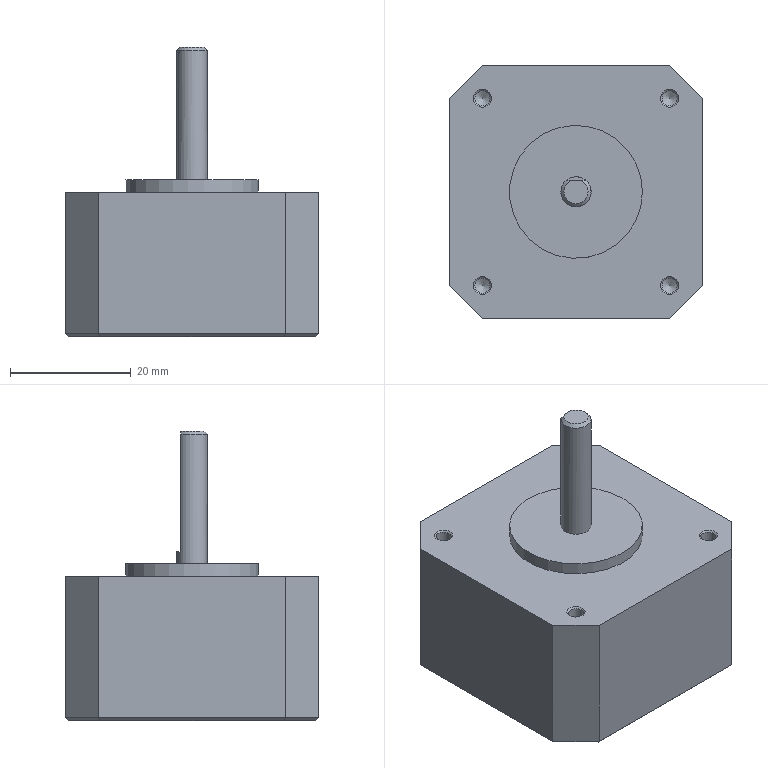Component | NX | DJZ_16_MOTOR | 2 solids | 38 faces | volume 41787 mm3 | plane 23 | cone 9 | cylinder 6 | commonest cylinder face diameters 2.5 x4 5 x1 22 x1